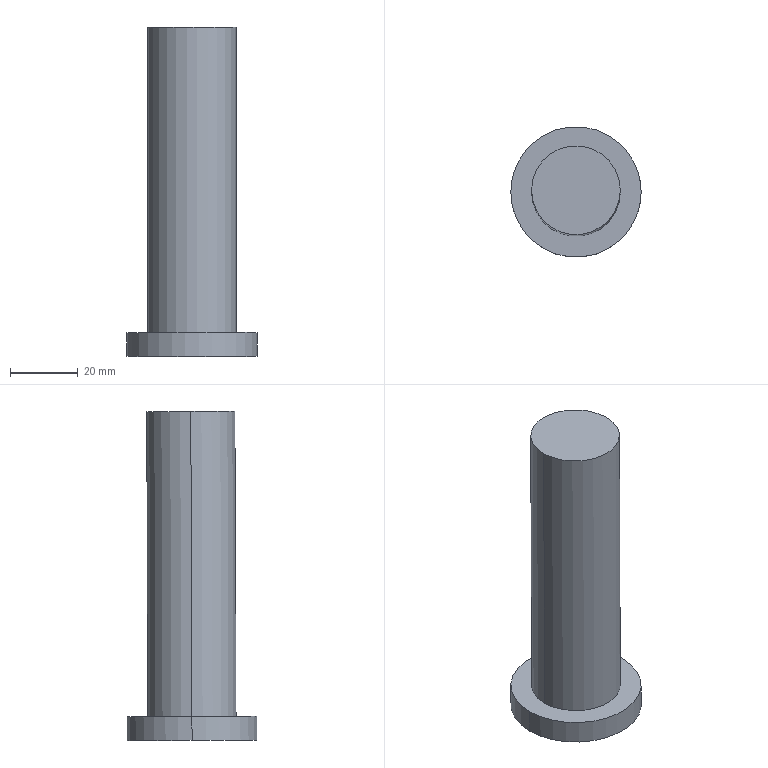Component | SolidWorks | RehabilitationChair-18-9-2 | 1 solid | 7 faces | box 38.39 x 38.41 x 96.94 mm | volume 56263 mm3 | cylinder 4 | plane 3 | commonest cylinder face diameters 26.129 x2 38.385 x2
STEP:
#1=COLOUR_RGB('',0.7922,0.8196,0.9333);
#2=FILL_AREA_STYLE_COLOUR('',#1);
#3=FILL_AREA_STYLE('',(#2));
#4=SURFACE_STYLE_FILL_AREA(#3);
#5=SURFACE_SIDE_STYLE('',(#4));
#6=SURFACE_STYLE_USAGE(.BOTH.,#5);
#7=PRESENTATION_STYLE_ASSIGNMENT((#6));
#8=CARTESIAN_POINT('',(12.204,15.288,16.735));
#9=VERTEX_POINT('',#8);
#10=CARTESIAN_POINT('',(13.232,15.288,16.735));
#11=VERTEX_POINT('',#10);
#12=CARTESIAN_POINT('',(12.718,15.288,16.735));
#13=DIRECTION('',(-0.0003323,0.003798,1.));
#14=DIRECTION('',(-1.,-0.00000716,-0.0003323));
#15=AXIS2_PLACEMENT_3D('',#12,#13,#14);
#16=CIRCLE('',#15,0.5144);
#17=EDGE_CURVE('',#9,#11,#16,.T.);
#18=ORIENTED_EDGE('',*,*,#17,.F.);
#19=CARTESIAN_POINT('',(12.205,15.275,13.199));
#20=VERTEX_POINT('',#19);
#21=CARTESIAN_POINT('',(12.204,15.288,16.784));
#22=DIRECTION('',(0.0003323,-0.003798,-1.));
#23=VECTOR('',#22,39.37);
#24=LINE('',#21,#23);
#25=EDGE_CURVE('',#9,#20,#24,.T.);
#26=ORIENTED_EDGE('',*,*,#25,.T.);
#27=CARTESIAN_POINT('',(13.233,15.275,13.199));
#28=VERTEX_POINT('',#27);
#29=CARTESIAN_POINT('',(12.719,15.275,13.199));
#30=DIRECTION('',(0.0003323,-0.003798,-1.));
#31=DIRECTION('',(1.,0.00000716,0.0003323));
#32=AXIS2_PLACEMENT_3D('',#29,#30,#31);
#33=CIRCLE('',#32,0.5144);
#34=EDGE_CURVE('',#28,#20,#33,.T.);
#35=ORIENTED_EDGE('',*,*,#34,.F.);
#36=CARTESIAN_POINT('',(13.232,15.288,16.784));
#37=DIRECTION('',(0.0003323,-0.003798,-1.));
#38=VECTOR('',#37,39.37);
#39=LINE('',#36,#38);
#40=EDGE_CURVE('',#11,#28,#39,.T.);
#41=ORIENTED_EDGE('',*,*,#40,.F.);
#42=EDGE_LOOP('',(#18,#26,#35,#41));
#43=FACE_OUTER_BOUND('',#42,.T.);
#44=CARTESIAN_POINT('',(12.718,15.288,16.784));
#45=DIRECTION('',(0.0003323,-0.003798,-1.));
#46=DIRECTION('',(1.,0.00000716,0.0003323));
#47=AXIS2_PLACEMENT_3D('',#44,#45,#46);
#48=CYLINDRICAL_SURFACE('',#47,0.5144);
#49=ADVANCED_FACE('',(#43),#48,.T.);
#50=CARTESIAN_POINT('',(13.475,15.274,12.923));
#51=VERTEX_POINT('',#50);
#52=CARTESIAN_POINT('',(11.964,15.274,12.923));
#53=VERTEX_POINT('',#52);
#54=CARTESIAN_POINT('',(12.719,15.274,12.923));
#55=DIRECTION('',(0.0003323,-0.003798,-1.));
#56=DIRECTION('',(1.,0.00000716,0.0003323));
#57=AXIS2_PLACEMENT_3D('',#54,#55,#56);
#58=CIRCLE('',#57,0.7556);
#59=EDGE_CURVE('',#51,#53,#58,.T.);
#60=ORIENTED_EDGE('',*,*,#59,.F.);
#61=CARTESIAN_POINT('',(13.475,15.275,13.199));
#62=VERTEX_POINT('',#61);
#63=CARTESIAN_POINT('',(13.475,15.274,12.923));
#64=DIRECTION('',(-0.0003323,0.003798,1.));
#65=VECTOR('',#64,39.37);
#66=LINE('',#63,#65);
#67=EDGE_CURVE('',#51,#62,#66,.T.);
#68=ORIENTED_EDGE('',*,*,#67,.T.);
#69=CARTESIAN_POINT('',(11.964,15.275,13.198));
#70=VERTEX_POINT('',#69);
#71=CARTESIAN_POINT('',(12.719,15.275,13.199));
#72=DIRECTION('',(0.0003323,-0.003798,-1.));
#73=DIRECTION('',(1.,0.00000716,0.0003323));
#74=AXIS2_PLACEMENT_3D('',#71,#72,#73);
#75=CIRCLE('',#74,0.7556);
#76=EDGE_CURVE('',#62,#70,#75,.T.);
#77=ORIENTED_EDGE('',*,*,#76,.T.);
#78=CARTESIAN_POINT('',(11.964,15.274,12.923));
#79=DIRECTION('',(-0.0003323,0.003798,1.));
#80=VECTOR('',#79,39.37);
#81=LINE('',#78,#80);
#82=EDGE_CURVE('',#53,#70,#81,.T.);
#83=ORIENTED_EDGE('',*,*,#82,.F.);
#84=EDGE_LOOP('',(#60,#68,#77,#83));
#85=FACE_OUTER_BOUND('',#84,.T.);
#86=CARTESIAN_POINT('',(12.719,15.274,12.923));
#87=DIRECTION('',(-0.0003323,0.003798,1.));
#88=DIRECTION('',(-1.,-0.00000716,-0.0003323));
#89=AXIS2_PLACEMENT_3D('',#86,#87,#88);
#90=CYLINDRICAL_SURFACE('',#89,0.7556);
#91=ADVANCED_FACE('',(#85),#90,.T.);
#92=ORIENTED_EDGE('',*,*,#67,.F.);
#93=CARTESIAN_POINT('',(12.719,15.274,12.923));
#94=DIRECTION('',(0.0003323,-0.003798,-1.));
#95=DIRECTION('',(1.,0.00000716,0.0003323));
#96=AXIS2_PLACEMENT_3D('',#93,#94,#95);
#97=CIRCLE('',#96,0.7556);
#98=EDGE_CURVE('',#53,#51,#97,.T.);
#99=ORIENTED_EDGE('',*,*,#98,.F.);
#100=ORIENTED_EDGE('',*,*,#82,.T.);
#101=CARTESIAN_POINT('',(12.719,15.275,13.199));
#102=DIRECTION('',(0.0003323,-0.003798,-1.));
#103=DIRECTION('',(1.,0.00000716,0.0003323));
#104=AXIS2_PLACEMENT_3D('',#101,#102,#103);
#105=CIRCLE('',#104,0.7556);
#106=EDGE_CURVE('',#70,#62,#105,.T.);
#107=ORIENTED_EDGE('',*,*,#106,.T.);
#108=EDGE_LOOP('',(#92,#99,#100,#107));
#109=FACE_OUTER_BOUND('',#108,.T.);
#110=CARTESIAN_POINT('',(12.719,15.274,12.923));
#111=DIRECTION('',(-0.0003323,0.003798,1.));
#112=DIRECTION('',(-1.,-0.00000716,-0.0003323));
#113=AXIS2_PLACEMENT_3D('',#110,#111,#112);
#114=CYLINDRICAL_SURFACE('',#113,0.7556);
#115=ADVANCED_FACE('',(#109),#114,.T.);
#116=ORIENTED_EDGE('',*,*,#98,.T.);
#117=ORIENTED_EDGE('',*,*,#59,.T.);
#118=EDGE_LOOP('',(#116,#117));
#119=FACE_OUTER_BOUND('',#118,.T.);
#120=CARTESIAN_POINT('',(12.719,15.274,12.923));
#121=DIRECTION('',(0.0003323,-0.003798,-1.));
#122=DIRECTION('',(1.,0.00000716,0.0003323));
#123=AXIS2_PLACEMENT_3D('',#120,#121,#122);
#124=PLANE('',#123);
#125=ADVANCED_FACE('',(#119),#124,.T.);
#126=ORIENTED_EDGE('',*,*,#34,.T.);
#127=CARTESIAN_POINT('',(12.719,15.275,13.199));
#128=DIRECTION('',(0.0003323,-0.003798,-1.));
#129=DIRECTION('',(1.,0.00000716,0.0003323));
#130=AXIS2_PLACEMENT_3D('',#127,#128,#129);
#131=CIRCLE('',#130,0.5144);
#132=EDGE_CURVE('',#20,#28,#131,.T.);
#133=ORIENTED_EDGE('',*,*,#132,.T.);
#134=EDGE_LOOP('',(#126,#133));
#135=FACE_BOUND('',#134,.T.);
#136=ORIENTED_EDGE('',*,*,#106,.F.);
#137=ORIENTED_EDGE('',*,*,#76,.F.);
#138=EDGE_LOOP('',(#136,#137));
#139=FACE_OUTER_BOUND('',#138,.T.);
#140=CARTESIAN_POINT('',(12.719,15.275,13.199));
#141=DIRECTION('',(0.0003323,-0.003798,-1.));
#142=DIRECTION('',(1.,0.00000716,0.0003323));
#143=AXIS2_PLACEMENT_3D('',#140,#141,#142);
#144=PLANE('',#143);
#145=ADVANCED_FACE('',(#135,#139),#144,.F.);
#146=CARTESIAN_POINT('',(12.718,15.288,16.735));
#147=DIRECTION('',(-0.0003323,0.003798,1.));
#148=DIRECTION('',(-1.,-0.00000716,-0.0003323));
#149=AXIS2_PLACEMENT_3D('',#146,#147,#148);
#150=CIRCLE('',#149,0.5144);
#151=EDGE_CURVE('',#11,#9,#150,.T.);
#152=ORIENTED_EDGE('',*,*,#151,.T.);
#153=ORIENTED_EDGE('',*,*,#17,.T.);
#154=EDGE_LOOP('',(#152,#153));
#155=FACE_OUTER_BOUND('',#154,.T.);
#156=CARTESIAN_POINT('',(12.718,15.288,16.735));
#157=DIRECTION('',(-0.0003323,0.003798,1.));
#158=DIRECTION('',(-0.08715,-0.9962,0.003755));
#159=AXIS2_PLACEMENT_3D('',#156,#157,#158);
#160=PLANE('',#159);
#161=ADVANCED_FACE('',(#155),#160,.T.);
#162=ORIENTED_EDGE('',*,*,#25,.F.);
#163=ORIENTED_EDGE('',*,*,#151,.F.);
#164=ORIENTED_EDGE('',*,*,#40,.T.);
#165=ORIENTED_EDGE('',*,*,#132,.F.);
#166=EDGE_LOOP('',(#162,#163,#164,#165));
#167=FACE_OUTER_BOUND('',#166,.T.);
#168=CARTESIAN_POINT('',(12.718,15.288,16.784));
#169=DIRECTION('',(0.0003323,-0.003798,-1.));
#170=DIRECTION('',(1.,0.00000716,0.0003323));
#171=AXIS2_PLACEMENT_3D('',#168,#169,#170);
#172=CYLINDRICAL_SURFACE('',#171,0.5144);
#173=ADVANCED_FACE('',(#167),#172,.T.);
#174=CLOSED_SHELL('',(#49,#91,#115,#125,#145,#161,#173));
#175=MANIFOLD_SOLID_BREP('',#174);
#176=STYLED_ITEM('',(#7),#175);
#177=PRESENTATION_LAYER_ASSIGNMENT('','',(#176));
#178=(LENGTH_UNIT()NAMED_UNIT(*)SI_UNIT($,.METRE.));
#179=LENGTH_MEASURE_WITH_UNIT(LENGTH_MEASURE(0.0254),#178);
#180=DIMENSIONAL_EXPONENTS(1.,0.,0.,0.,0.,0.,0.);
#181=(CONVERSION_BASED_UNIT('',#179)LENGTH_UNIT()NAMED_UNIT(#180));
#182=UNCERTAINTY_MEASURE_WITH_UNIT(LENGTH_MEASURE(0.00001),#181,'','');
#183=(NAMED_UNIT(*)PLANE_ANGLE_UNIT()SI_UNIT($,.RADIAN.));
#184=(NAMED_UNIT(*)SI_UNIT($,.STERADIAN.)SOLID_ANGLE_UNIT());
#185=(GEOMETRIC_REPRESENTATION_CONTEXT(3)GLOBAL_UNCERTAINTY_ASSIGNED_CONTEXT((#182))GLOBAL_UNIT_ASSIGNED_CONTEXT((#181,#183,#184))REPRESENTATION_CONTEXT('',''));
#186=MECHANICAL_DESIGN_GEOMETRIC_PRESENTATION_REPRESENTATION('',(#176),#185);
#187=CARTESIAN_POINT('',(0.,0.,0.));
#188=DIRECTION('',(0.,0.,1.));
#189=DIRECTION('',(1.,0.,0.));
#190=AXIS2_PLACEMENT_3D('',#187,#188,#189);
#191=(LENGTH_UNIT()NAMED_UNIT(*)SI_UNIT($,.METRE.));
#192=LENGTH_MEASURE_WITH_UNIT(LENGTH_MEASURE(0.0254),#191);
#193=DIMENSIONAL_EXPONENTS(1.,0.,0.,0.,0.,0.,0.);
#194=(CONVERSION_BASED_UNIT('',#192)LENGTH_UNIT()NAMED_UNIT(#193));
#195=UNCERTAINTY_MEASURE_WITH_UNIT(LENGTH_MEASURE(0.00001),#194,'','');
#196=(NAMED_UNIT(*)PLANE_ANGLE_UNIT()SI_UNIT($,.RADIAN.));
#197=(NAMED_UNIT(*)SI_UNIT($,.STERADIAN.)SOLID_ANGLE_UNIT());
#198=(GEOMETRIC_REPRESENTATION_CONTEXT(3)GLOBAL_UNCERTAINTY_ASSIGNED_CONTEXT((#195))GLOBAL_UNIT_ASSIGNED_CONTEXT((#194,#196,#197))REPRESENTATION_CONTEXT('',''));
#199=ADVANCED_BREP_SHAPE_REPRESENTATION('',(#175,#190),#198);